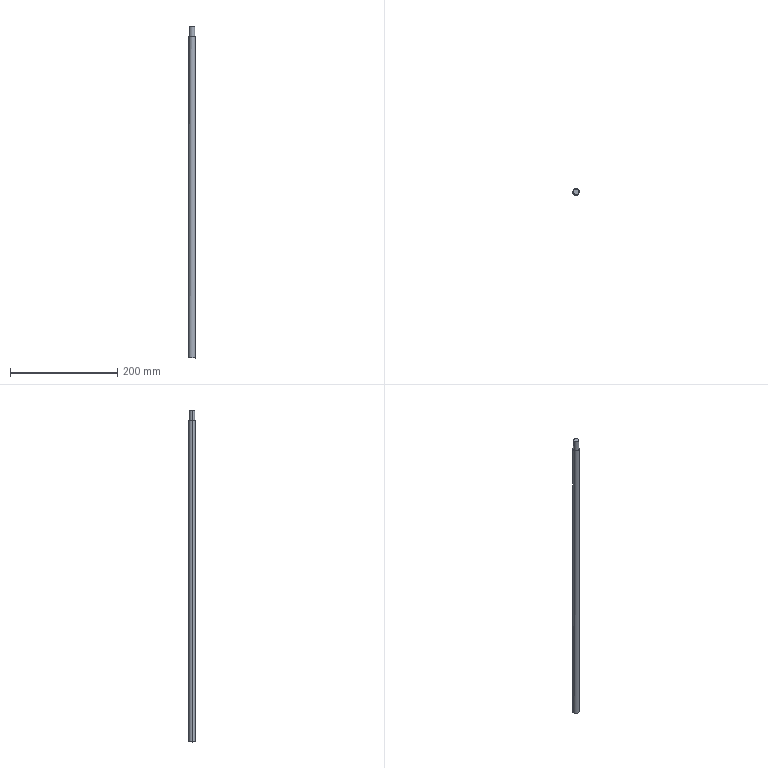Component | SolidWorks | ArmTelescopicCylinderPistonRod-1 | 1 solid | 7 faces | box 12.65 x 12 x 620.01 mm | volume 69429 mm3 | cylinder 4 | plane 3 | commonest cylinder face diameters 10 x2 12 x2
build123d program:
from build123d import *

# Parameters (mm, degrees)
SKETCH1_R           = 6
BOSS_EXTRUDE1_DEPTH = 600
SKETCH2_R           = 5
BOSS_EXTRUDE2_DEPTH = 20


with BuildPart() as part:
    # Sketch1 → Boss-Extrude1 (new body)
    with BuildSketch(Plane(origin=(0, 0, 0), x_dir=(1, 0, 0), z_dir=(0, 1, 0))):
        with Locations(Location((0, 0, 0), (0, 0, 270))):
            Circle(SKETCH1_R)
    extrude(amount=BOSS_EXTRUDE1_DEPTH)

    # Sketch2 → Boss-Extrude2 (add)
    with BuildSketch(Plane(origin=(0, 600, 0), x_dir=(1, 0, 0), z_dir=(0, 1, 0))):
        with Locations(Location((0, 0, 0), (0, 0, 270))):
            Circle(SKETCH2_R)
    extrude(amount=BOSS_EXTRUDE2_DEPTH)


solid = part.part

# Placed as in the assembly
solid = solid.moved(Location((-96.441, 871.583, 444.721), (-90.571, 83.808, -179.426)))
STEP:
#1=COLOUR_RGB('',0.7922,0.8196,0.9333);
#2=FILL_AREA_STYLE_COLOUR('',#1);
#3=FILL_AREA_STYLE('',(#2));
#4=SURFACE_STYLE_FILL_AREA(#3);
#5=SURFACE_SIDE_STYLE('',(#4));
#6=SURFACE_STYLE_USAGE(.BOTH.,#5);
#7=PRESENTATION_STYLE_ASSIGNMENT((#6));
#8=CARTESIAN_POINT('',(-3.576,34.345,41.918));
#9=VERTEX_POINT('',#8);
#10=CARTESIAN_POINT('',(-3.965,34.284,41.918));
#11=VERTEX_POINT('',#10);
#12=CARTESIAN_POINT('',(-3.771,34.314,41.918));
#13=DIRECTION('',(0.00108,0.,1.));
#14=DIRECTION('',(0.9879,0.155,-0.001067));
#15=AXIS2_PLACEMENT_3D('',#12,#13,#14);
#16=CIRCLE('',#15,0.1969);
#17=EDGE_CURVE('',#9,#11,#16,.T.);
#18=ORIENTED_EDGE('',*,*,#17,.F.);
#19=CARTESIAN_POINT('',(-3.577,34.345,41.131));
#20=VERTEX_POINT('',#19);
#21=CARTESIAN_POINT('',(-3.576,34.345,41.918));
#22=DIRECTION('',(-0.00108,-0.,-1.));
#23=VECTOR('',#22,39.37);
#24=LINE('',#21,#23);
#25=EDGE_CURVE('',#9,#20,#24,.T.);
#26=ORIENTED_EDGE('',*,*,#25,.T.);
#27=CARTESIAN_POINT('',(-3.966,34.284,41.131));
#28=VERTEX_POINT('',#27);
#29=CARTESIAN_POINT('',(-3.771,34.314,41.131));
#30=DIRECTION('',(0.00108,0.,1.));
#31=DIRECTION('',(0.9879,0.155,-0.001067));
#32=AXIS2_PLACEMENT_3D('',#29,#30,#31);
#33=CIRCLE('',#32,0.1969);
#34=EDGE_CURVE('',#20,#28,#33,.T.);
#35=ORIENTED_EDGE('',*,*,#34,.T.);
#36=CARTESIAN_POINT('',(-3.965,34.284,41.918));
#37=DIRECTION('',(-0.00108,-0.,-1.));
#38=VECTOR('',#37,39.37);
#39=LINE('',#36,#38);
#40=EDGE_CURVE('',#11,#28,#39,.T.);
#41=ORIENTED_EDGE('',*,*,#40,.F.);
#42=EDGE_LOOP('',(#18,#26,#35,#41));
#43=FACE_OUTER_BOUND('',#42,.T.);
#44=CARTESIAN_POINT('',(-3.771,34.314,41.918));
#45=DIRECTION('',(-0.00108,-0.,-1.));
#46=DIRECTION('',(-0.9879,-0.155,0.001067));
#47=AXIS2_PLACEMENT_3D('',#44,#45,#46);
#48=CYLINDRICAL_SURFACE('',#47,0.1969);
#49=ADVANCED_FACE('',(#43),#48,.T.);
#50=CARTESIAN_POINT('',(-3.538,34.351,41.13));
#51=VERTEX_POINT('',#50);
#52=CARTESIAN_POINT('',(-4.005,34.278,41.131));
#53=VERTEX_POINT('',#52);
#54=CARTESIAN_POINT('',(-3.771,34.314,41.131));
#55=DIRECTION('',(0.00108,0.,1.));
#56=DIRECTION('',(0.9879,0.155,-0.001067));
#57=AXIS2_PLACEMENT_3D('',#54,#55,#56);
#58=CIRCLE('',#57,0.2362);
#59=EDGE_CURVE('',#51,#53,#58,.T.);
#60=ORIENTED_EDGE('',*,*,#59,.F.);
#61=CARTESIAN_POINT('',(-3.564,34.351,17.508));
#62=VERTEX_POINT('',#61);
#63=CARTESIAN_POINT('',(-3.538,34.351,41.13));
#64=DIRECTION('',(-0.00108,-0.,-1.));
#65=VECTOR('',#64,39.37);
#66=LINE('',#63,#65);
#67=EDGE_CURVE('',#51,#62,#66,.T.);
#68=ORIENTED_EDGE('',*,*,#67,.T.);
#69=CARTESIAN_POINT('',(-4.03,34.278,17.509));
#70=VERTEX_POINT('',#69);
#71=CARTESIAN_POINT('',(-3.797,34.314,17.509));
#72=DIRECTION('',(0.00108,0.,1.));
#73=DIRECTION('',(0.9879,0.155,-0.001067));
#74=AXIS2_PLACEMENT_3D('',#71,#72,#73);
#75=CIRCLE('',#74,0.2362);
#76=EDGE_CURVE('',#62,#70,#75,.T.);
#77=ORIENTED_EDGE('',*,*,#76,.T.);
#78=CARTESIAN_POINT('',(-4.005,34.278,41.131));
#79=DIRECTION('',(-0.00108,-0.,-1.));
#80=VECTOR('',#79,39.37);
#81=LINE('',#78,#80);
#82=EDGE_CURVE('',#53,#70,#81,.T.);
#83=ORIENTED_EDGE('',*,*,#82,.F.);
#84=EDGE_LOOP('',(#60,#68,#77,#83));
#85=FACE_OUTER_BOUND('',#84,.T.);
#86=CARTESIAN_POINT('',(-3.771,34.314,41.131));
#87=DIRECTION('',(-0.00108,-0.,-1.));
#88=DIRECTION('',(-0.9879,-0.155,0.001067));
#89=AXIS2_PLACEMENT_3D('',#86,#87,#88);
#90=CYLINDRICAL_SURFACE('',#89,0.2362);
#91=ADVANCED_FACE('',(#85),#90,.T.);
#92=ORIENTED_EDGE('',*,*,#67,.F.);
#93=CARTESIAN_POINT('',(-3.771,34.314,41.131));
#94=DIRECTION('',(0.00108,0.,1.));
#95=DIRECTION('',(0.9879,0.155,-0.001067));
#96=AXIS2_PLACEMENT_3D('',#93,#94,#95);
#97=CIRCLE('',#96,0.2362);
#98=EDGE_CURVE('',#53,#51,#97,.T.);
#99=ORIENTED_EDGE('',*,*,#98,.F.);
#100=ORIENTED_EDGE('',*,*,#82,.T.);
#101=CARTESIAN_POINT('',(-3.797,34.314,17.509));
#102=DIRECTION('',(0.00108,0.,1.));
#103=DIRECTION('',(0.9879,0.155,-0.001067));
#104=AXIS2_PLACEMENT_3D('',#101,#102,#103);
#105=CIRCLE('',#104,0.2362);
#106=EDGE_CURVE('',#70,#62,#105,.T.);
#107=ORIENTED_EDGE('',*,*,#106,.T.);
#108=EDGE_LOOP('',(#92,#99,#100,#107));
#109=FACE_OUTER_BOUND('',#108,.T.);
#110=CARTESIAN_POINT('',(-3.771,34.314,41.131));
#111=DIRECTION('',(-0.00108,-0.,-1.));
#112=DIRECTION('',(-0.9879,-0.155,0.001067));
#113=AXIS2_PLACEMENT_3D('',#110,#111,#112);
#114=CYLINDRICAL_SURFACE('',#113,0.2362);
#115=ADVANCED_FACE('',(#109),#114,.T.);
#116=CARTESIAN_POINT('',(-3.771,34.314,41.131));
#117=DIRECTION('',(0.00108,0.,1.));
#118=DIRECTION('',(0.9879,0.155,-0.001067));
#119=AXIS2_PLACEMENT_3D('',#116,#117,#118);
#120=CIRCLE('',#119,0.1969);
#121=EDGE_CURVE('',#28,#20,#120,.T.);
#122=ORIENTED_EDGE('',*,*,#121,.F.);
#123=ORIENTED_EDGE('',*,*,#34,.F.);
#124=EDGE_LOOP('',(#122,#123));
#125=FACE_BOUND('',#124,.T.);
#126=ORIENTED_EDGE('',*,*,#98,.T.);
#127=ORIENTED_EDGE('',*,*,#59,.T.);
#128=EDGE_LOOP('',(#126,#127));
#129=FACE_OUTER_BOUND('',#128,.T.);
#130=CARTESIAN_POINT('',(-3.771,34.314,41.131));
#131=DIRECTION('',(0.00108,0.,1.));
#132=DIRECTION('',(0.9879,0.155,-0.001067));
#133=AXIS2_PLACEMENT_3D('',#130,#131,#132);
#134=PLANE('',#133);
#135=ADVANCED_FACE('',(#125,#129),#134,.T.);
#136=ORIENTED_EDGE('',*,*,#106,.F.);
#137=ORIENTED_EDGE('',*,*,#76,.F.);
#138=EDGE_LOOP('',(#136,#137));
#139=FACE_OUTER_BOUND('',#138,.T.);
#140=CARTESIAN_POINT('',(-3.797,34.314,17.509));
#141=DIRECTION('',(0.00108,0.,1.));
#142=DIRECTION('',(0.9879,0.155,-0.001067));
#143=AXIS2_PLACEMENT_3D('',#140,#141,#142);
#144=PLANE('',#143);
#145=ADVANCED_FACE('',(#139),#144,.F.);
#146=ORIENTED_EDGE('',*,*,#25,.F.);
#147=CARTESIAN_POINT('',(-3.771,34.314,41.918));
#148=DIRECTION('',(0.00108,0.,1.));
#149=DIRECTION('',(0.9879,0.155,-0.001067));
#150=AXIS2_PLACEMENT_3D('',#147,#148,#149);
#151=CIRCLE('',#150,0.1969);
#152=EDGE_CURVE('',#11,#9,#151,.T.);
#153=ORIENTED_EDGE('',*,*,#152,.F.);
#154=ORIENTED_EDGE('',*,*,#40,.T.);
#155=ORIENTED_EDGE('',*,*,#121,.T.);
#156=EDGE_LOOP('',(#146,#153,#154,#155));
#157=FACE_OUTER_BOUND('',#156,.T.);
#158=CARTESIAN_POINT('',(-3.771,34.314,41.918));
#159=DIRECTION('',(-0.00108,-0.,-1.));
#160=DIRECTION('',(-0.9879,-0.155,0.001067));
#161=AXIS2_PLACEMENT_3D('',#158,#159,#160);
#162=CYLINDRICAL_SURFACE('',#161,0.1969);
#163=ADVANCED_FACE('',(#157),#162,.T.);
#164=ORIENTED_EDGE('',*,*,#152,.T.);
#165=ORIENTED_EDGE('',*,*,#17,.T.);
#166=EDGE_LOOP('',(#164,#165));
#167=FACE_OUTER_BOUND('',#166,.T.);
#168=CARTESIAN_POINT('',(-3.771,34.314,41.918));
#169=DIRECTION('',(0.00108,0.,1.));
#170=DIRECTION('',(0.9879,0.155,-0.001067));
#171=AXIS2_PLACEMENT_3D('',#168,#169,#170);
#172=PLANE('',#171);
#173=ADVANCED_FACE('',(#167),#172,.T.);
#174=CLOSED_SHELL('',(#49,#91,#115,#135,#145,#163,#173));
#175=MANIFOLD_SOLID_BREP('',#174);
#176=STYLED_ITEM('',(#7),#175);
#177=PRESENTATION_LAYER_ASSIGNMENT('','',(#176));
#178=CARTESIAN_POINT('',(0.,0.,0.));
#179=DIRECTION('',(0.,0.,1.));
#180=DIRECTION('',(1.,0.,0.));
#181=AXIS2_PLACEMENT_3D('',#178,#179,#180);
#182=(LENGTH_UNIT()NAMED_UNIT(*)SI_UNIT($,.METRE.));
#183=LENGTH_MEASURE_WITH_UNIT(LENGTH_MEASURE(0.0254),#182);
#184=DIMENSIONAL_EXPONENTS(1.,0.,0.,0.,0.,0.,0.);
#185=(CONVERSION_BASED_UNIT('',#183)LENGTH_UNIT()NAMED_UNIT(#184));
#186=UNCERTAINTY_MEASURE_WITH_UNIT(LENGTH_MEASURE(0.00001),#185,'','');
#187=(NAMED_UNIT(*)PLANE_ANGLE_UNIT()SI_UNIT($,.RADIAN.));
#188=(NAMED_UNIT(*)SI_UNIT($,.STERADIAN.)SOLID_ANGLE_UNIT());
#189=(GEOMETRIC_REPRESENTATION_CONTEXT(3)GLOBAL_UNCERTAINTY_ASSIGNED_CONTEXT((#186))GLOBAL_UNIT_ASSIGNED_CONTEXT((#185,#187,#188))REPRESENTATION_CONTEXT('',''));
#190=ADVANCED_BREP_SHAPE_REPRESENTATION('',(#175,#181),#189);
#191=(LENGTH_UNIT()NAMED_UNIT(*)SI_UNIT($,.METRE.));
#192=LENGTH_MEASURE_WITH_UNIT(LENGTH_MEASURE(0.0254),#191);
#193=DIMENSIONAL_EXPONENTS(1.,0.,0.,0.,0.,0.,0.);
#194=(CONVERSION_BASED_UNIT('',#192)LENGTH_UNIT()NAMED_UNIT(#193));
#195=UNCERTAINTY_MEASURE_WITH_UNIT(LENGTH_MEASURE(0.00001),#194,'','');
#196=(NAMED_UNIT(*)PLANE_ANGLE_UNIT()SI_UNIT($,.RADIAN.));
#197=(NAMED_UNIT(*)SI_UNIT($,.STERADIAN.)SOLID_ANGLE_UNIT());
#198=(GEOMETRIC_REPRESENTATION_CONTEXT(3)GLOBAL_UNCERTAINTY_ASSIGNED_CONTEXT((#195))GLOBAL_UNIT_ASSIGNED_CONTEXT((#194,#196,#197))REPRESENTATION_CONTEXT('',''));
#199=MECHANICAL_DESIGN_GEOMETRIC_PRESENTATION_REPRESENTATION('',(#176),#198);